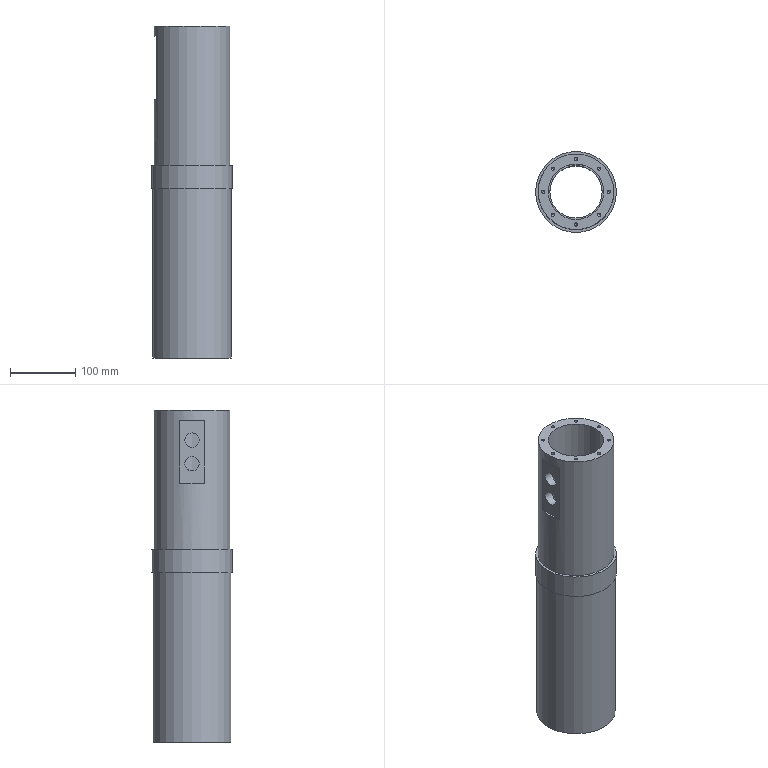Component | NX | CH3404_8_2-1 | 1 solid | 39 faces | volume 2752462 mm3 | cylinder 19 | plane 12 | cone 8 | commonest cylinder face diameters 5 x8 22.2 x2 116 x1 124 x1 120 x1 101 x1 95 x1 80 x1